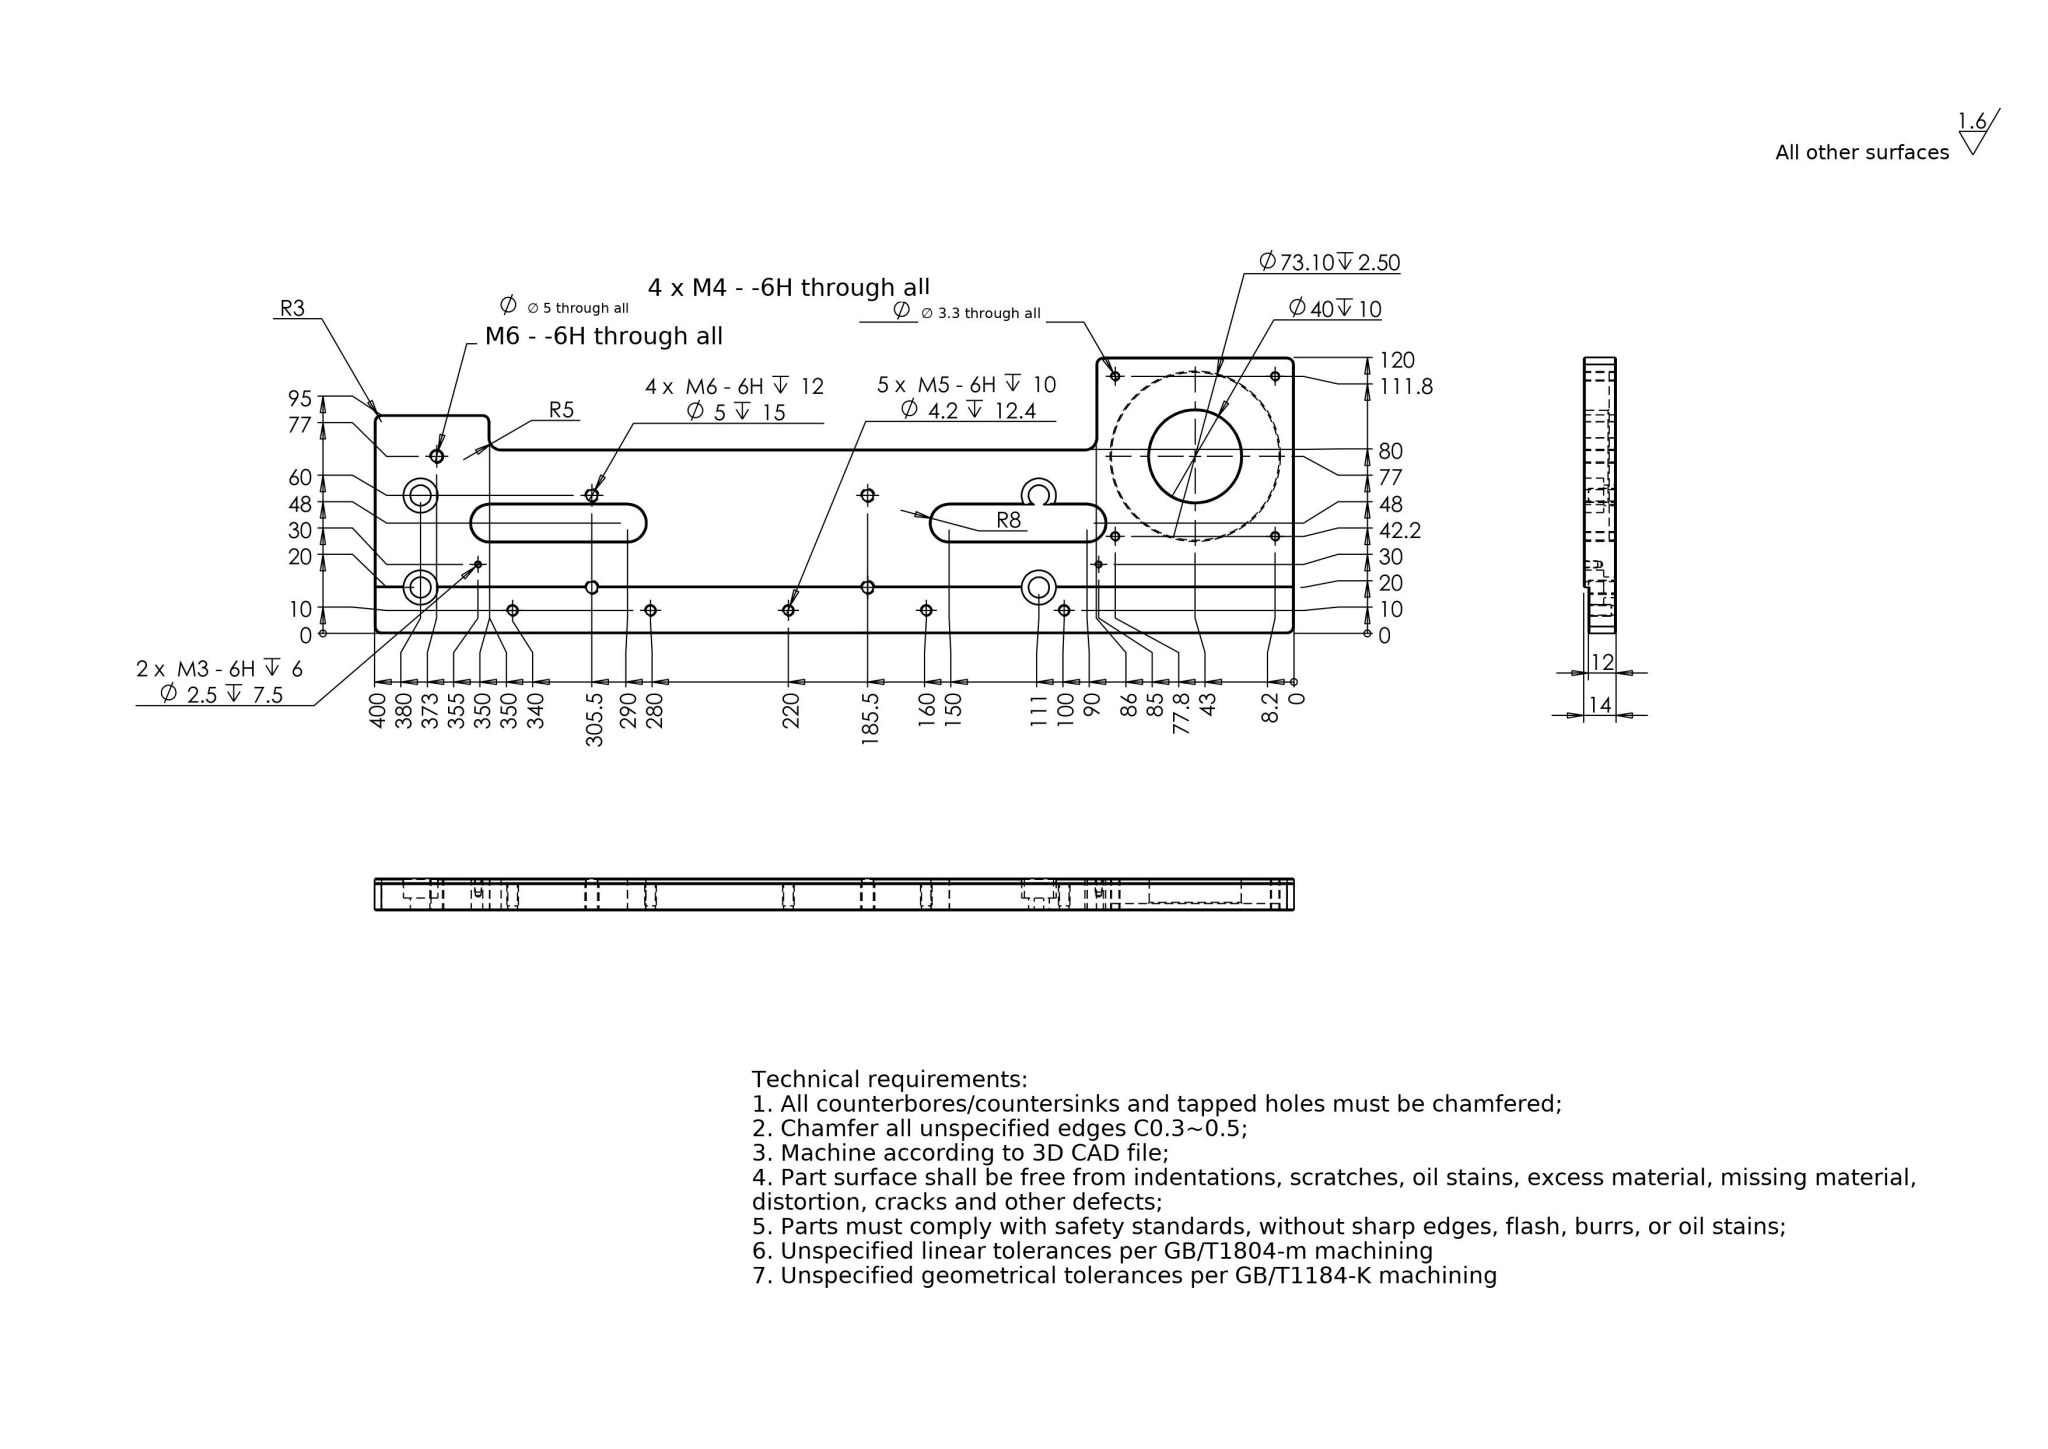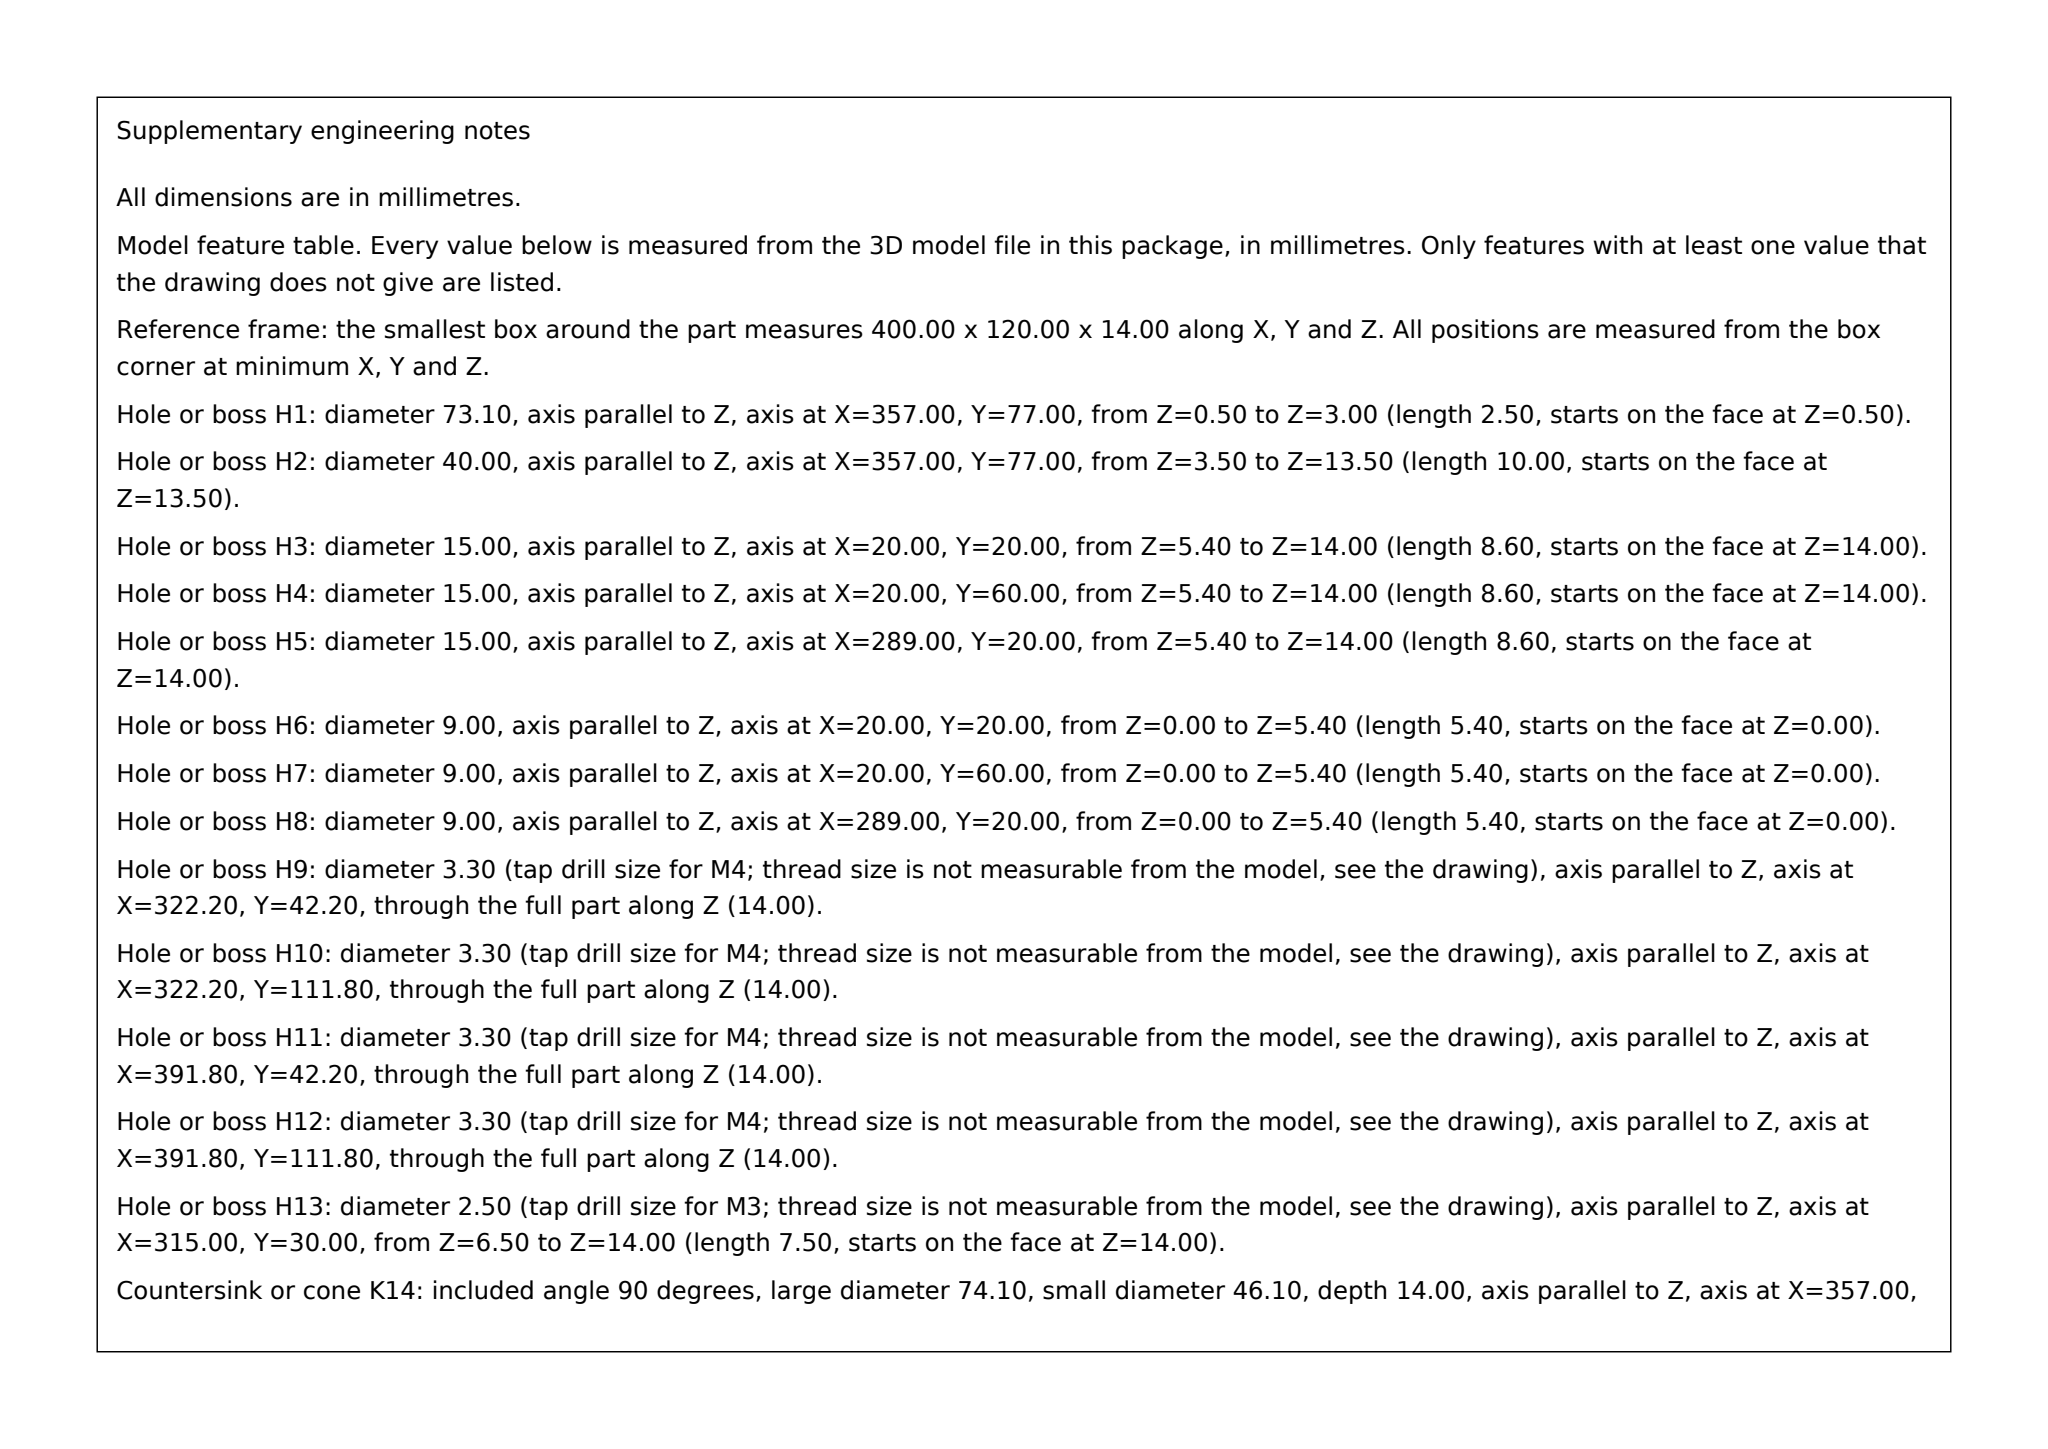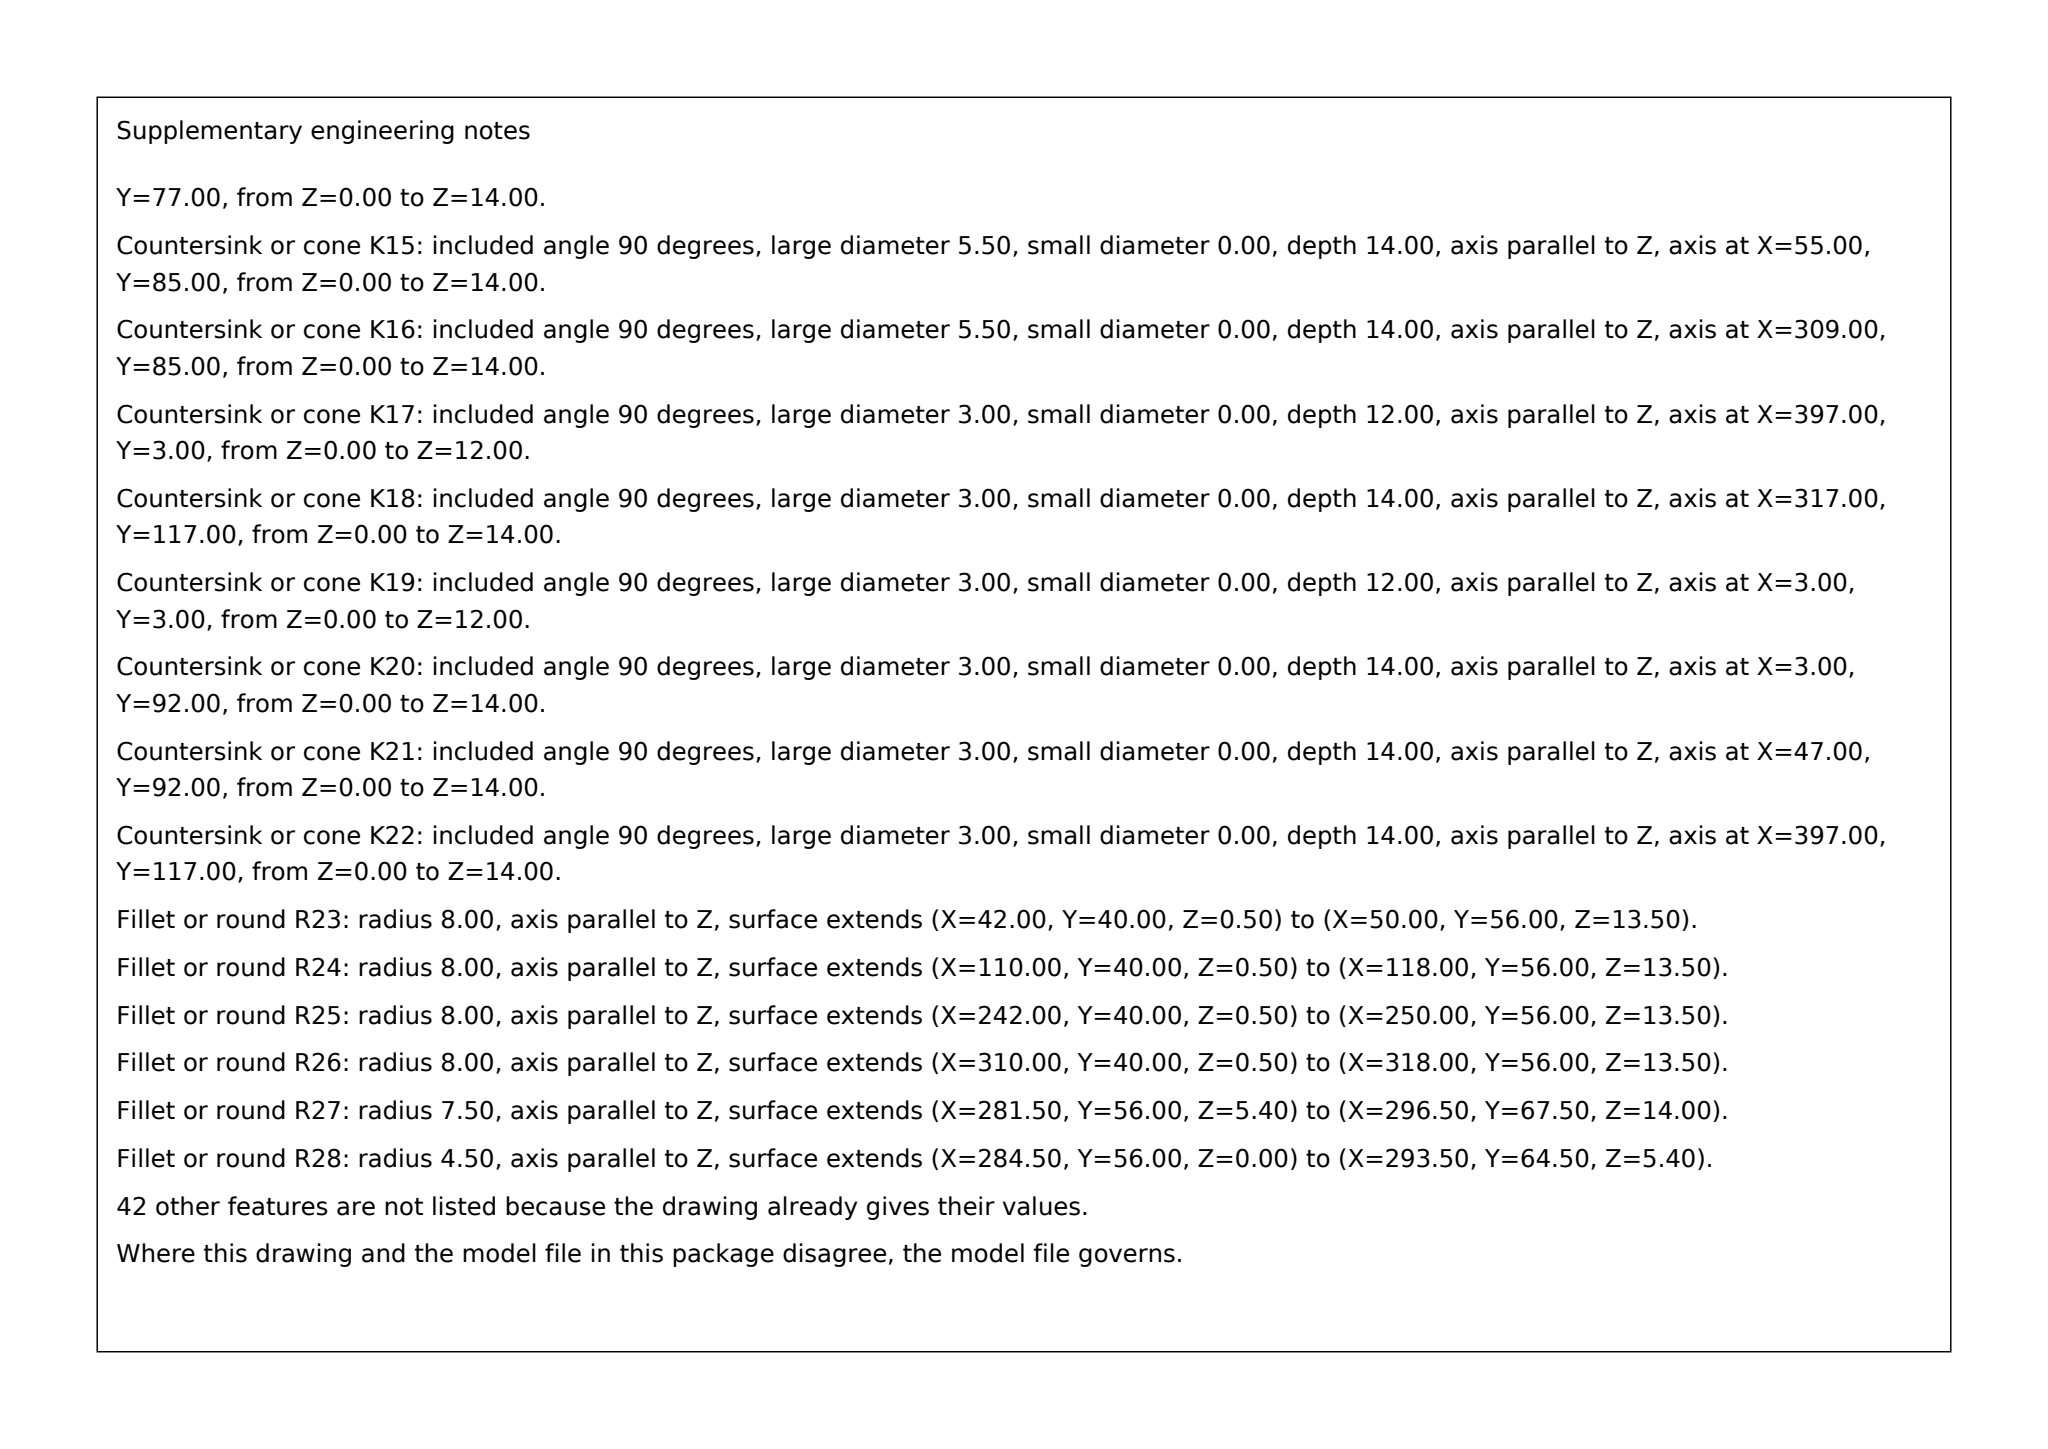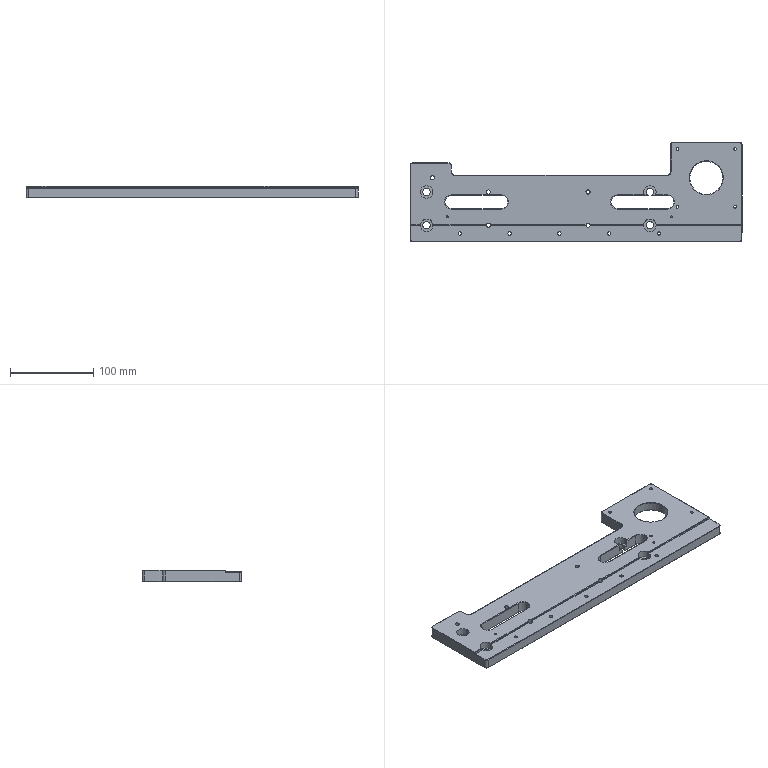Part | SolidWorks | mm | 1 solid | 165 faces | box 400 x 120 x 14 mm | volume 421735 mm3 | cylinder 68 | plane 59 | cone 38 | commonest cylinder face diameters 4.2 x10 5 x10 15 x9 9 x9 3.3 x8 16 x6 6 x6 2.5 x4